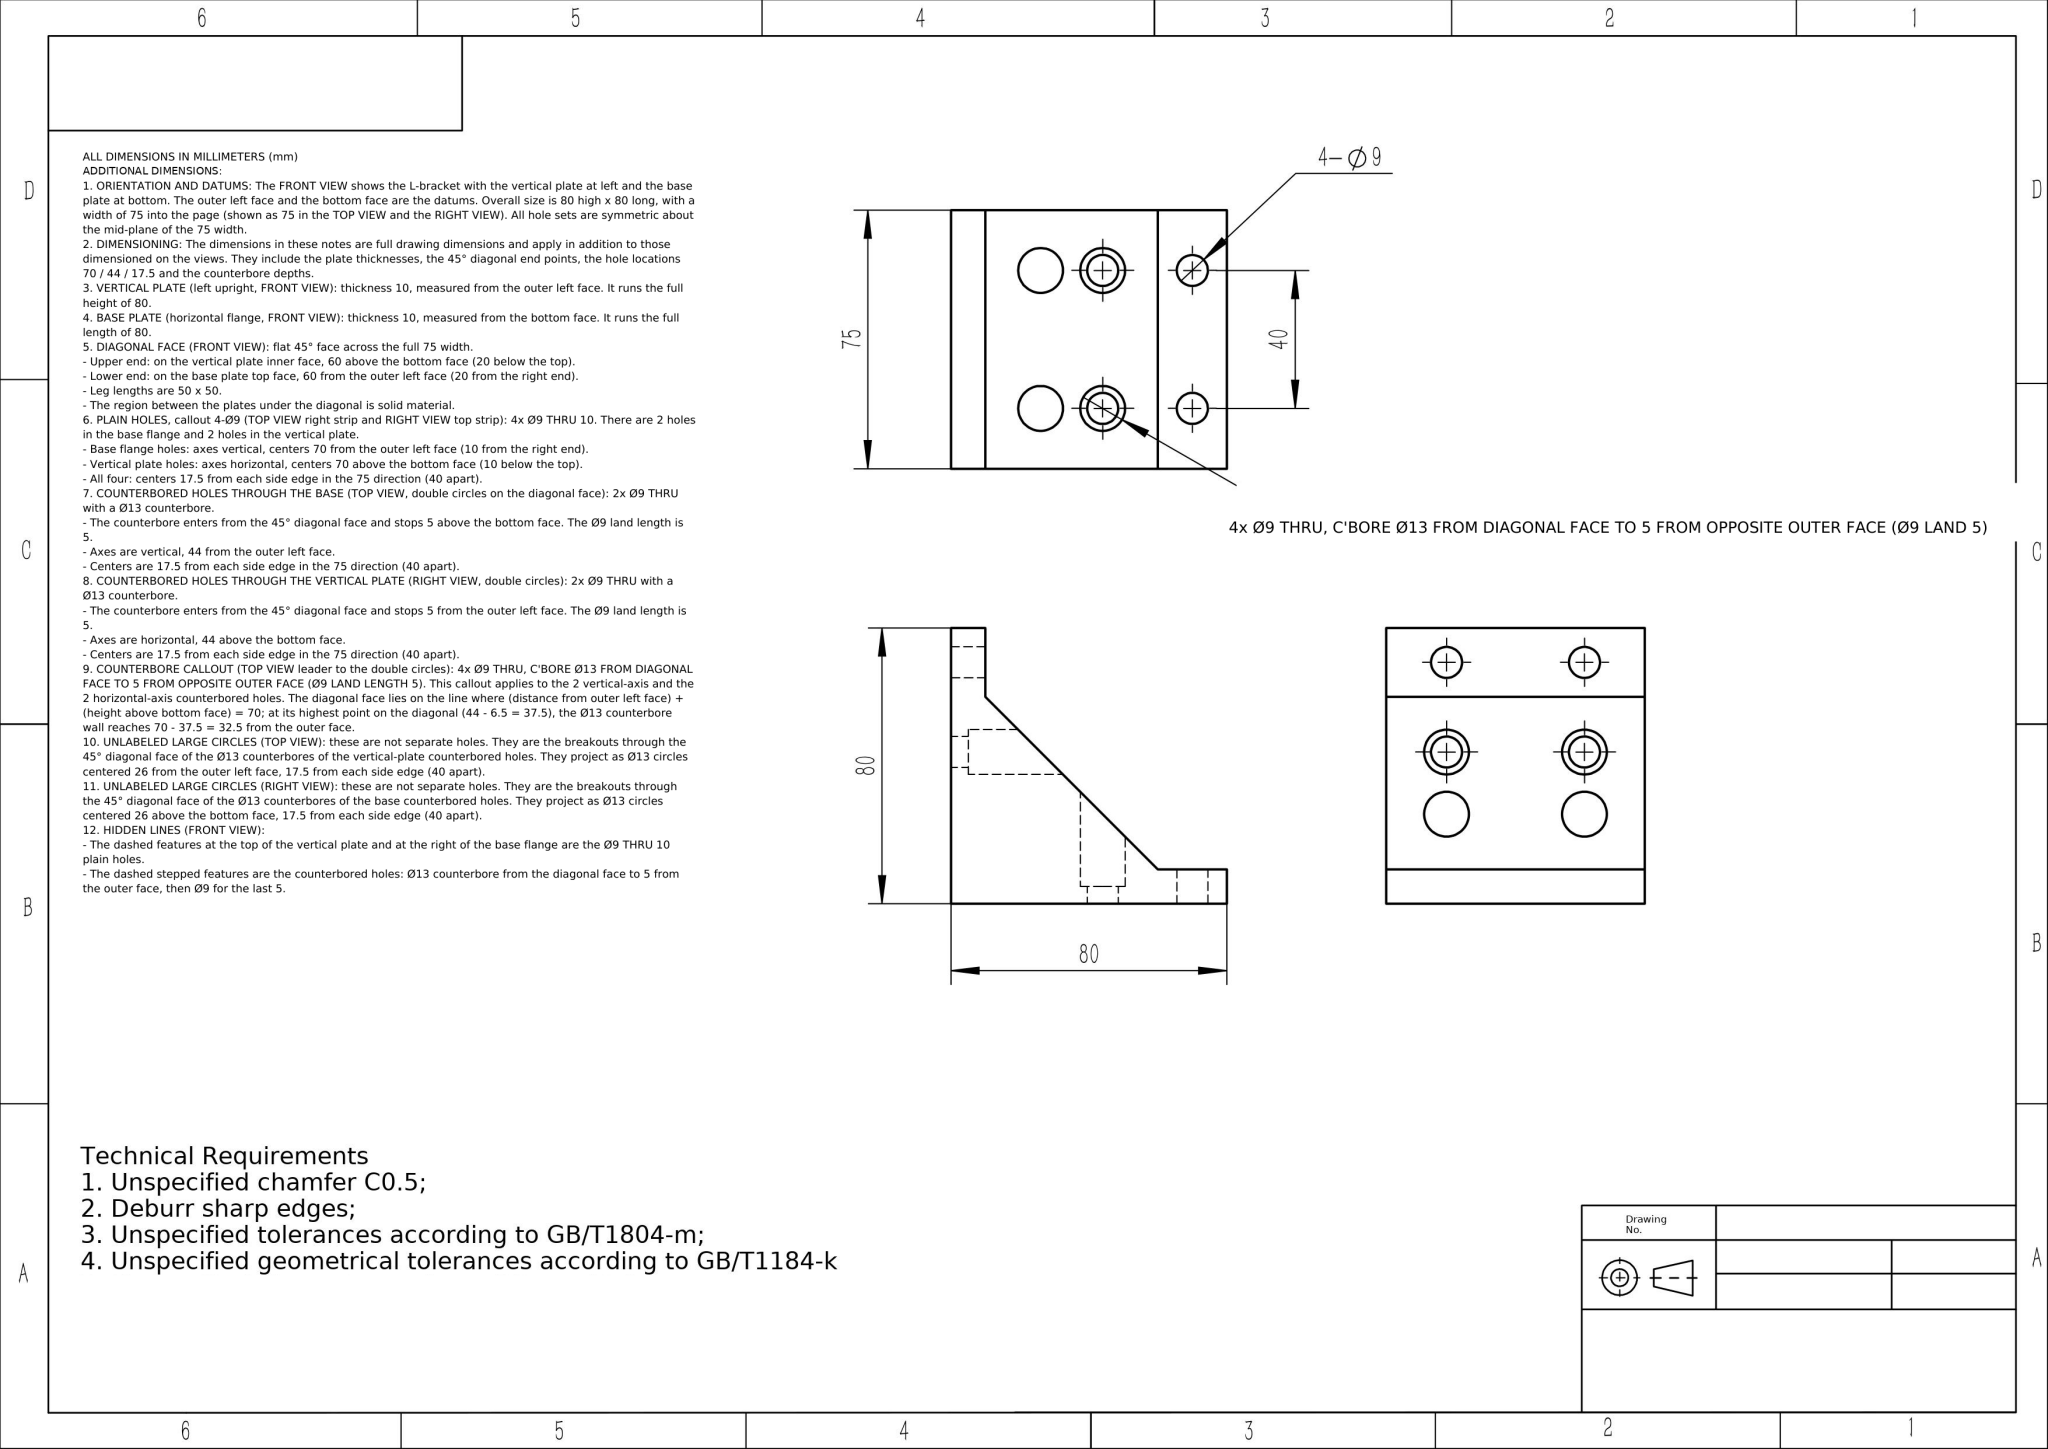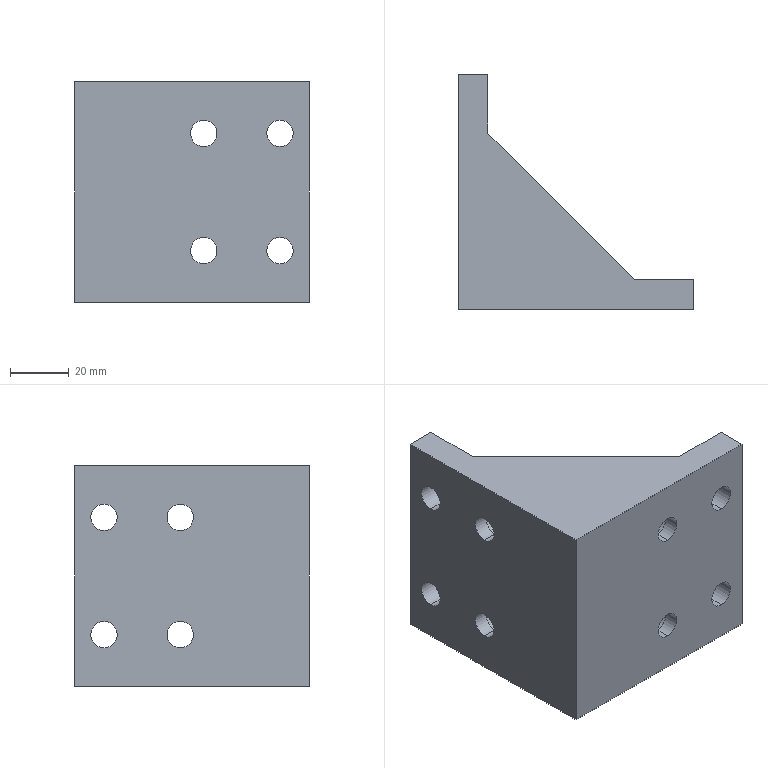Part | NX | mm | 1 solid | 37 faces | box 80 x 80 x 75 mm | volume 191284 mm3 | cylinder 24 | plane 13 | commonest cylinder face diameters 9 x16 13 x8